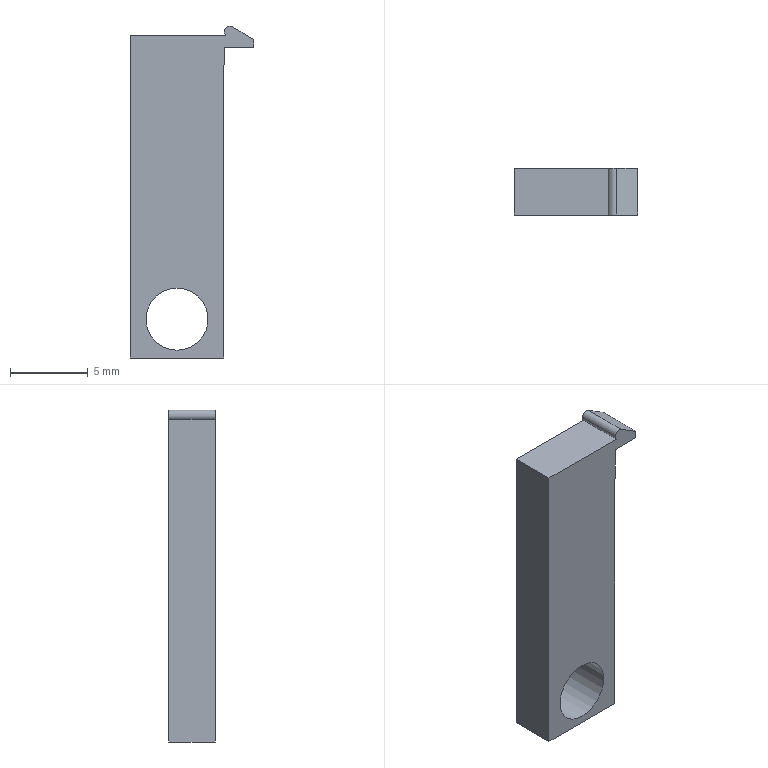Component | NX | SHEJI-WAIGUAN-3 | 1 solid | 12 faces | box 7.93 x 3 x 21.38 mm | volume 342 mm3 | plane 10 | cylinder 2 | commonest cylinder face diameters 0.707 x1 4 x1
STEP:
#1=CARTESIAN_POINT('',(0.,0.,0.));
#2=DIRECTION('',(0.,0.,1.));
#3=DIRECTION('',(1.,0.,0.));
#4=AXIS2_PLACEMENT_3D('',#1,#2,#3);
#5=CARTESIAN_POINT('',(-72.,-1.5,27.));
#6=VERTEX_POINT('',#5);
#7=CARTESIAN_POINT('',(-72.,-1.5,11.));
#8=VERTEX_POINT('',#7);
#9=CARTESIAN_POINT('',(-72.,-1.5,27.));
#10=DIRECTION('',(0.,0.,-1.));
#11=VECTOR('',#10,1.);
#12=LINE('',#9,#11);
#13=CARTESIAN_POINT('',(-72.,1.5,27.));
#14=DIRECTION('',(-1.,0.,0.));
#15=DIRECTION('',(0.,0.,-1.));
#16=AXIS2_PLACEMENT_3D('',#13,#14,#15);
#17=PLANE('',#16);
#18=CARTESIAN_POINT('',(0.,3.));
#19=DIRECTION('',(1.,0.));
#20=VECTOR('',#19,1.);
#21=LINE('',#18,#20);
#22=(GEOMETRIC_REPRESENTATION_CONTEXT(2)PARAMETRIC_REPRESENTATION_CONTEXT()REPRESENTATION_CONTEXT('',''));
#23=DEFINITIONAL_REPRESENTATION('',(#21),#22);
#24=PCURVE('',#17,#23);
#25=CARTESIAN_POINT('',(-71.606,-1.5,32.023));
#26=DIRECTION('',(0.,1.,0.));
#27=DIRECTION('',(0.,0.,-1.));
#28=AXIS2_PLACEMENT_3D('',#25,#26,#27);
#29=PLANE('',#28);
#30=CARTESIAN_POINT('',(5.023,0.3939));
#31=DIRECTION('',(1.,0.));
#32=VECTOR('',#31,1.);
#33=LINE('',#30,#32);
#34=(GEOMETRIC_REPRESENTATION_CONTEXT(2)PARAMETRIC_REPRESENTATION_CONTEXT()REPRESENTATION_CONTEXT('',''));
#35=DEFINITIONAL_REPRESENTATION('',(#33),#34);
#36=PCURVE('',#29,#35);
#37=SURFACE_CURVE('',#12,(#24,#36),.PCURVE_S1.);
#38=EDGE_CURVE('',#6,#8,#37,.T.);
#39=ORIENTED_EDGE('',*,*,#38,.T.);
#40=CARTESIAN_POINT('',(-72.,1.5,11.));
#41=VERTEX_POINT('',#40);
#42=CARTESIAN_POINT('',(-72.,1.5,11.));
#43=DIRECTION('',(0.,-1.,0.));
#44=VECTOR('',#43,1.);
#45=LINE('',#42,#44);
#46=CARTESIAN_POINT('',(16.,0.));
#47=DIRECTION('',(0.,1.));
#48=VECTOR('',#47,1.);
#49=LINE('',#46,#48);
#50=(GEOMETRIC_REPRESENTATION_CONTEXT(2)PARAMETRIC_REPRESENTATION_CONTEXT()REPRESENTATION_CONTEXT('',''));
#51=DEFINITIONAL_REPRESENTATION('',(#49),#50);
#52=PCURVE('',#17,#51);
#53=CARTESIAN_POINT('',(-72.,1.5,11.));
#54=DIRECTION('',(0.,0.,1.));
#55=DIRECTION('',(-1.,0.,0.));
#56=AXIS2_PLACEMENT_3D('',#53,#54,#55);
#57=PLANE('',#56);
#58=CARTESIAN_POINT('',(0.,0.));
#59=DIRECTION('',(0.,1.));
#60=VECTOR('',#59,1.);
#61=LINE('',#58,#60);
#62=(GEOMETRIC_REPRESENTATION_CONTEXT(2)PARAMETRIC_REPRESENTATION_CONTEXT()REPRESENTATION_CONTEXT('',''));
#63=DEFINITIONAL_REPRESENTATION('',(#61),#62);
#64=PCURVE('',#57,#63);
#65=SURFACE_CURVE('',#45,(#52,#64),.PCURVE_S1.);
#66=EDGE_CURVE('',#41,#8,#65,.T.);
#67=ORIENTED_EDGE('',*,*,#66,.F.);
#68=CARTESIAN_POINT('',(-72.,1.5,27.));
#69=VERTEX_POINT('',#68);
#70=CARTESIAN_POINT('',(-72.,1.5,27.));
#71=DIRECTION('',(0.,0.,-1.));
#72=VECTOR('',#71,1.);
#73=LINE('',#70,#72);
#74=CARTESIAN_POINT('',(0.,0.));
#75=DIRECTION('',(1.,0.));
#76=VECTOR('',#75,1.);
#77=LINE('',#74,#76);
#78=(GEOMETRIC_REPRESENTATION_CONTEXT(2)PARAMETRIC_REPRESENTATION_CONTEXT()REPRESENTATION_CONTEXT('',''));
#79=DEFINITIONAL_REPRESENTATION('',(#77),#78);
#80=PCURVE('',#17,#79);
#81=CARTESIAN_POINT('',(-71.606,1.5,32.023));
#82=DIRECTION('',(0.,1.,0.));
#83=DIRECTION('',(0.,0.,-1.));
#84=AXIS2_PLACEMENT_3D('',#81,#82,#83);
#85=PLANE('',#84);
#86=CARTESIAN_POINT('',(5.023,0.3939));
#87=DIRECTION('',(1.,0.));
#88=VECTOR('',#87,1.);
#89=LINE('',#86,#88);
#90=(GEOMETRIC_REPRESENTATION_CONTEXT(2)PARAMETRIC_REPRESENTATION_CONTEXT()REPRESENTATION_CONTEXT('',''));
#91=DEFINITIONAL_REPRESENTATION('',(#89),#90);
#92=PCURVE('',#85,#91);
#93=SURFACE_CURVE('',#73,(#80,#92),.PCURVE_S1.);
#94=EDGE_CURVE('',#69,#41,#93,.T.);
#95=ORIENTED_EDGE('',*,*,#94,.F.);
#96=CARTESIAN_POINT('',(-72.,1.5,27.));
#97=DIRECTION('',(0.,-1.,0.));
#98=VECTOR('',#97,1.);
#99=LINE('',#96,#98);
#100=CARTESIAN_POINT('',(0.,0.));
#101=DIRECTION('',(0.,1.));
#102=VECTOR('',#101,1.);
#103=LINE('',#100,#102);
#104=(GEOMETRIC_REPRESENTATION_CONTEXT(2)PARAMETRIC_REPRESENTATION_CONTEXT()REPRESENTATION_CONTEXT('',''));
#105=DEFINITIONAL_REPRESENTATION('',(#103),#104);
#106=PCURVE('',#17,#105);
#107=CARTESIAN_POINT('',(-71.968,1.5,31.));
#108=DIRECTION('',(-1.,0.,0.008057));
#109=DIRECTION('',(-0.008057,0.,-1.));
#110=AXIS2_PLACEMENT_3D('',#107,#108,#109);
#111=PLANE('',#110);
#112=CARTESIAN_POINT('',(4.,0.));
#113=DIRECTION('',(0.,1.));
#114=VECTOR('',#113,1.);
#115=LINE('',#112,#114);
#116=(GEOMETRIC_REPRESENTATION_CONTEXT(2)PARAMETRIC_REPRESENTATION_CONTEXT()REPRESENTATION_CONTEXT('',''));
#117=DEFINITIONAL_REPRESENTATION('',(#115),#116);
#118=PCURVE('',#111,#117);
#119=SURFACE_CURVE('',#99,(#106,#118),.PCURVE_S1.);
#120=EDGE_CURVE('',#69,#6,#119,.T.);
#121=ORIENTED_EDGE('',*,*,#120,.T.);
#122=EDGE_LOOP('',(#39,#67,#95,#121));
#123=FACE_BOUND('',#122,.T.);
#124=ADVANCED_FACE('',(#123),#17,.F.);
#125=CARTESIAN_POINT('',(-78.,-1.5,11.));
#126=VERTEX_POINT('',#125);
#127=CARTESIAN_POINT('',(-72.,-1.5,11.));
#128=DIRECTION('',(-1.,0.,0.));
#129=VECTOR('',#128,1.);
#130=LINE('',#127,#129);
#131=CARTESIAN_POINT('',(0.,3.));
#132=DIRECTION('',(1.,0.));
#133=VECTOR('',#132,1.);
#134=LINE('',#131,#133);
#135=(GEOMETRIC_REPRESENTATION_CONTEXT(2)PARAMETRIC_REPRESENTATION_CONTEXT()REPRESENTATION_CONTEXT('',''));
#136=DEFINITIONAL_REPRESENTATION('',(#134),#135);
#137=PCURVE('',#57,#136);
#138=CARTESIAN_POINT('',(21.023,0.3939));
#139=DIRECTION('',(0.,1.));
#140=VECTOR('',#139,1.);
#141=LINE('',#138,#140);
#142=(GEOMETRIC_REPRESENTATION_CONTEXT(2)PARAMETRIC_REPRESENTATION_CONTEXT()REPRESENTATION_CONTEXT('',''));
#143=DEFINITIONAL_REPRESENTATION('',(#141),#142);
#144=PCURVE('',#29,#143);
#145=SURFACE_CURVE('',#130,(#137,#144),.PCURVE_S1.);
#146=EDGE_CURVE('',#8,#126,#145,.T.);
#147=ORIENTED_EDGE('',*,*,#146,.T.);
#148=CARTESIAN_POINT('',(-78.,1.5,11.));
#149=VERTEX_POINT('',#148);
#150=CARTESIAN_POINT('',(-78.,1.5,11.));
#151=DIRECTION('',(0.,-1.,0.));
#152=VECTOR('',#151,1.);
#153=LINE('',#150,#152);
#154=CARTESIAN_POINT('',(6.,0.));
#155=DIRECTION('',(0.,1.));
#156=VECTOR('',#155,1.);
#157=LINE('',#154,#156);
#158=(GEOMETRIC_REPRESENTATION_CONTEXT(2)PARAMETRIC_REPRESENTATION_CONTEXT()REPRESENTATION_CONTEXT('',''));
#159=DEFINITIONAL_REPRESENTATION('',(#157),#158);
#160=PCURVE('',#57,#159);
#161=CARTESIAN_POINT('',(-78.,1.5,31.));
#162=DIRECTION('',(1.,0.,0.));
#163=DIRECTION('',(0.,0.,1.));
#164=AXIS2_PLACEMENT_3D('',#161,#162,#163);
#165=PLANE('',#164);
#166=CARTESIAN_POINT('',(-20.,0.));
#167=DIRECTION('',(0.,1.));
#168=VECTOR('',#167,1.);
#169=LINE('',#166,#168);
#170=(GEOMETRIC_REPRESENTATION_CONTEXT(2)PARAMETRIC_REPRESENTATION_CONTEXT()REPRESENTATION_CONTEXT('',''));
#171=DEFINITIONAL_REPRESENTATION('',(#169),#170);
#172=PCURVE('',#165,#171);
#173=SURFACE_CURVE('',#153,(#160,#172),.PCURVE_S1.);
#174=EDGE_CURVE('',#149,#126,#173,.T.);
#175=ORIENTED_EDGE('',*,*,#174,.F.);
#176=CARTESIAN_POINT('',(-72.,1.5,11.));
#177=DIRECTION('',(-1.,0.,0.));
#178=VECTOR('',#177,1.);
#179=LINE('',#176,#178);
#180=CARTESIAN_POINT('',(0.,0.));
#181=DIRECTION('',(1.,0.));
#182=VECTOR('',#181,1.);
#183=LINE('',#180,#182);
#184=(GEOMETRIC_REPRESENTATION_CONTEXT(2)PARAMETRIC_REPRESENTATION_CONTEXT()REPRESENTATION_CONTEXT('',''));
#185=DEFINITIONAL_REPRESENTATION('',(#183),#184);
#186=PCURVE('',#57,#185);
#187=CARTESIAN_POINT('',(21.023,0.3939));
#188=DIRECTION('',(0.,1.));
#189=VECTOR('',#188,1.);
#190=LINE('',#187,#189);
#191=(GEOMETRIC_REPRESENTATION_CONTEXT(2)PARAMETRIC_REPRESENTATION_CONTEXT()REPRESENTATION_CONTEXT('',''));
#192=DEFINITIONAL_REPRESENTATION('',(#190),#191);
#193=PCURVE('',#85,#192);
#194=SURFACE_CURVE('',#179,(#186,#193),.PCURVE_S1.);
#195=EDGE_CURVE('',#41,#149,#194,.T.);
#196=ORIENTED_EDGE('',*,*,#195,.F.);
#197=ORIENTED_EDGE('',*,*,#66,.T.);
#198=EDGE_LOOP('',(#147,#175,#196,#197));
#199=FACE_BOUND('',#198,.T.);
#200=ADVANCED_FACE('',(#199),#57,.F.);
#201=CARTESIAN_POINT('',(-78.,-1.5,31.776));
#202=VERTEX_POINT('',#201);
#203=CARTESIAN_POINT('',(-78.,-1.5,31.));
#204=DIRECTION('',(0.,0.,1.));
#205=VECTOR('',#204,1.);
#206=LINE('',#203,#205);
#207=CARTESIAN_POINT('',(0.,3.));
#208=DIRECTION('',(1.,0.));
#209=VECTOR('',#208,1.);
#210=LINE('',#207,#209);
#211=(GEOMETRIC_REPRESENTATION_CONTEXT(2)PARAMETRIC_REPRESENTATION_CONTEXT()REPRESENTATION_CONTEXT('',''));
#212=DEFINITIONAL_REPRESENTATION('',(#210),#211);
#213=PCURVE('',#165,#212);
#214=CARTESIAN_POINT('',(1.023,6.394));
#215=DIRECTION('',(-1.,0.));
#216=VECTOR('',#215,1.);
#217=LINE('',#214,#216);
#218=(GEOMETRIC_REPRESENTATION_CONTEXT(2)PARAMETRIC_REPRESENTATION_CONTEXT()REPRESENTATION_CONTEXT('',''));
#219=DEFINITIONAL_REPRESENTATION('',(#217),#218);
#220=PCURVE('',#29,#219);
#221=SURFACE_CURVE('',#206,(#213,#220),.PCURVE_S1.);
#222=EDGE_CURVE('',#126,#202,#221,.T.);
#223=ORIENTED_EDGE('',*,*,#222,.T.);
#224=CARTESIAN_POINT('',(-78.,1.5,31.776));
#225=VERTEX_POINT('',#224);
#226=CARTESIAN_POINT('',(-78.,1.5,31.776));
#227=DIRECTION('',(0.,-1.,0.));
#228=VECTOR('',#227,1.);
#229=LINE('',#226,#228);
#230=CARTESIAN_POINT('',(0.7762,0.));
#231=DIRECTION('',(0.,1.));
#232=VECTOR('',#231,1.);
#233=LINE('',#230,#232);
#234=(GEOMETRIC_REPRESENTATION_CONTEXT(2)PARAMETRIC_REPRESENTATION_CONTEXT()REPRESENTATION_CONTEXT('',''));
#235=DEFINITIONAL_REPRESENTATION('',(#233),#234);
#236=PCURVE('',#165,#235);
#237=CARTESIAN_POINT('',(-78.,1.5,31.776));
#238=DIRECTION('',(0.,0.,-1.));
#239=DIRECTION('',(1.,0.,0.));
#240=AXIS2_PLACEMENT_3D('',#237,#238,#239);
#241=PLANE('',#240);
#242=CARTESIAN_POINT('',(0.,0.));
#243=DIRECTION('',(0.,1.));
#244=VECTOR('',#243,1.);
#245=LINE('',#242,#244);
#246=(GEOMETRIC_REPRESENTATION_CONTEXT(2)PARAMETRIC_REPRESENTATION_CONTEXT()REPRESENTATION_CONTEXT('',''));
#247=DEFINITIONAL_REPRESENTATION('',(#245),#246);
#248=PCURVE('',#241,#247);
#249=SURFACE_CURVE('',#229,(#236,#248),.PCURVE_S1.);
#250=EDGE_CURVE('',#225,#202,#249,.T.);
#251=ORIENTED_EDGE('',*,*,#250,.F.);
#252=CARTESIAN_POINT('',(-78.,1.5,11.));
#253=DIRECTION('',(0.,0.,1.));
#254=VECTOR('',#253,1.);
#255=LINE('',#252,#254);
#256=CARTESIAN_POINT('',(-20.,0.));
#257=DIRECTION('',(1.,0.));
#258=VECTOR('',#257,1.);
#259=LINE('',#256,#258);
#260=(GEOMETRIC_REPRESENTATION_CONTEXT(2)PARAMETRIC_REPRESENTATION_CONTEXT()REPRESENTATION_CONTEXT('',''));
#261=DEFINITIONAL_REPRESENTATION('',(#259),#260);
#262=PCURVE('',#165,#261);
#263=CARTESIAN_POINT('',(21.023,6.394));
#264=DIRECTION('',(-1.,0.));
#265=VECTOR('',#264,1.);
#266=LINE('',#263,#265);
#267=(GEOMETRIC_REPRESENTATION_CONTEXT(2)PARAMETRIC_REPRESENTATION_CONTEXT()REPRESENTATION_CONTEXT('',''));
#268=DEFINITIONAL_REPRESENTATION('',(#266),#267);
#269=PCURVE('',#85,#268);
#270=SURFACE_CURVE('',#255,(#262,#269),.PCURVE_S1.);
#271=EDGE_CURVE('',#149,#225,#270,.T.);
#272=ORIENTED_EDGE('',*,*,#271,.F.);
#273=ORIENTED_EDGE('',*,*,#174,.T.);
#274=EDGE_LOOP('',(#223,#251,#272,#273));
#275=FACE_BOUND('',#274,.T.);
#276=ADVANCED_FACE('',(#275),#165,.F.);
#277=CARTESIAN_POINT('',(-71.859,-1.5,31.776));
#278=VERTEX_POINT('',#277);
#279=CARTESIAN_POINT('',(-78.,-1.5,31.776));
#280=DIRECTION('',(1.,0.,0.));
#281=VECTOR('',#280,1.);
#282=LINE('',#279,#281);
#283=CARTESIAN_POINT('',(0.,3.));
#284=DIRECTION('',(1.,0.));
#285=VECTOR('',#284,1.);
#286=LINE('',#283,#285);
#287=(GEOMETRIC_REPRESENTATION_CONTEXT(2)PARAMETRIC_REPRESENTATION_CONTEXT()REPRESENTATION_CONTEXT('',''));
#288=DEFINITIONAL_REPRESENTATION('',(#286),#287);
#289=PCURVE('',#241,#288);
#290=CARTESIAN_POINT('',(0.2472,6.394));
#291=DIRECTION('',(0.,-1.));
#292=VECTOR('',#291,1.);
#293=LINE('',#290,#292);
#294=(GEOMETRIC_REPRESENTATION_CONTEXT(2)PARAMETRIC_REPRESENTATION_CONTEXT()REPRESENTATION_CONTEXT('',''));
#295=DEFINITIONAL_REPRESENTATION('',(#293),#294);
#296=PCURVE('',#29,#295);
#297=SURFACE_CURVE('',#282,(#289,#296),.PCURVE_S1.);
#298=EDGE_CURVE('',#202,#278,#297,.T.);
#299=ORIENTED_EDGE('',*,*,#298,.T.);
#300=CARTESIAN_POINT('',(-71.859,1.5,31.776));
#301=VERTEX_POINT('',#300);
#302=CARTESIAN_POINT('',(-71.859,1.5,31.776));
#303=DIRECTION('',(0.,-1.,0.));
#304=VECTOR('',#303,1.);
#305=LINE('',#302,#304);
#306=CARTESIAN_POINT('',(6.141,-0.));
#307=DIRECTION('',(0.,1.));
#308=VECTOR('',#307,1.);
#309=LINE('',#306,#308);
#310=(GEOMETRIC_REPRESENTATION_CONTEXT(2)PARAMETRIC_REPRESENTATION_CONTEXT()REPRESENTATION_CONTEXT('',''));
#311=DEFINITIONAL_REPRESENTATION('',(#309),#310);
#312=PCURVE('',#241,#311);
#313=CARTESIAN_POINT('',(-71.606,1.5,32.023));
#314=DIRECTION('',(0.,-1.,0.));
#315=DIRECTION('',(0.,0.,1.));
#316=AXIS2_PLACEMENT_3D('',#313,#314,#315);
#317=CYLINDRICAL_SURFACE('',#316,0.3534);
#318=CARTESIAN_POINT('',(2.345,0.));
#319=DIRECTION('',(0.,1.));
#320=VECTOR('',#319,1.);
#321=LINE('',#318,#320);
#322=(GEOMETRIC_REPRESENTATION_CONTEXT(2)PARAMETRIC_REPRESENTATION_CONTEXT()REPRESENTATION_CONTEXT('',''));
#323=DEFINITIONAL_REPRESENTATION('',(#321),#322);
#324=PCURVE('',#317,#323);
#325=SURFACE_CURVE('',#305,(#312,#324),.PCURVE_S1.);
#326=EDGE_CURVE('',#301,#278,#325,.T.);
#327=ORIENTED_EDGE('',*,*,#326,.F.);
#328=CARTESIAN_POINT('',(-78.,1.5,31.776));
#329=DIRECTION('',(1.,0.,0.));
#330=VECTOR('',#329,1.);
#331=LINE('',#328,#330);
#332=CARTESIAN_POINT('',(0.,0.));
#333=DIRECTION('',(1.,0.));
#334=VECTOR('',#333,1.);
#335=LINE('',#332,#334);
#336=(GEOMETRIC_REPRESENTATION_CONTEXT(2)PARAMETRIC_REPRESENTATION_CONTEXT()REPRESENTATION_CONTEXT('',''));
#337=DEFINITIONAL_REPRESENTATION('',(#335),#336);
#338=PCURVE('',#241,#337);
#339=CARTESIAN_POINT('',(0.2472,6.394));
#340=DIRECTION('',(0.,-1.));
#341=VECTOR('',#340,1.);
#342=LINE('',#339,#341);
#343=(GEOMETRIC_REPRESENTATION_CONTEXT(2)PARAMETRIC_REPRESENTATION_CONTEXT()REPRESENTATION_CONTEXT('',''));
#344=DEFINITIONAL_REPRESENTATION('',(#342),#343);
#345=PCURVE('',#85,#344);
#346=SURFACE_CURVE('',#331,(#338,#345),.PCURVE_S1.);
#347=EDGE_CURVE('',#225,#301,#346,.T.);
#348=ORIENTED_EDGE('',*,*,#347,.F.);
#349=ORIENTED_EDGE('',*,*,#250,.T.);
#350=EDGE_LOOP('',(#299,#327,#348,#349));
#351=FACE_BOUND('',#350,.T.);
#352=ADVANCED_FACE('',(#351),#241,.F.);
#353=CARTESIAN_POINT('',(-71.421,-1.5,32.325));
#354=VERTEX_POINT('',#353);
#355=CARTESIAN_POINT('',(-71.606,-1.5,32.023));
#356=DIRECTION('',(0.,1.,0.));
#357=DIRECTION('',(-1.,0.,0.));
#358=AXIS2_PLACEMENT_3D('',#355,#356,#357);
#359=CIRCLE('',#358,0.3534);
#360=CARTESIAN_POINT('',(7.854,3.));
#361=DIRECTION('',(-1.,0.));
#362=VECTOR('',#361,1.);
#363=LINE('',#360,#362);
#364=(GEOMETRIC_REPRESENTATION_CONTEXT(2)PARAMETRIC_REPRESENTATION_CONTEXT()REPRESENTATION_CONTEXT('',''));
#365=DEFINITIONAL_REPRESENTATION('',(#363),#364);
#366=PCURVE('',#317,#365);
#367=CARTESIAN_POINT('',(0.,0.));
#368=DIRECTION('',(0.,1.));
#369=AXIS2_PLACEMENT_2D('',#367,#368);
#370=CIRCLE('',#369,0.3534);
#371=(GEOMETRIC_REPRESENTATION_CONTEXT(2)PARAMETRIC_REPRESENTATION_CONTEXT()REPRESENTATION_CONTEXT('',''));
#372=DEFINITIONAL_REPRESENTATION('',(#370),#371);
#373=PCURVE('',#29,#372);
#374=SURFACE_CURVE('',#359,(#366,#373),.PCURVE_S1.);
#375=EDGE_CURVE('',#278,#354,#374,.T.);
#376=ORIENTED_EDGE('',*,*,#375,.T.);
#377=CARTESIAN_POINT('',(-71.421,1.5,32.325));
#378=VERTEX_POINT('',#377);
#379=CARTESIAN_POINT('',(-71.421,1.5,32.325));
#380=DIRECTION('',(0.,-1.,0.));
#381=VECTOR('',#380,1.);
#382=LINE('',#379,#381);
#383=CARTESIAN_POINT('',(-0.5495,0.));
#384=DIRECTION('',(0.,1.));
#385=VECTOR('',#384,1.);
#386=LINE('',#383,#385);
#387=(GEOMETRIC_REPRESENTATION_CONTEXT(2)PARAMETRIC_REPRESENTATION_CONTEXT()REPRESENTATION_CONTEXT('',''));
#388=DEFINITIONAL_REPRESENTATION('',(#386),#387);
#389=PCURVE('',#317,#388);
#390=CARTESIAN_POINT('',(-71.421,1.5,32.325));
#391=DIRECTION('',(-0.5223,0.,-0.8528));
#392=DIRECTION('',(0.8528,0.,-0.5223));
#393=AXIS2_PLACEMENT_3D('',#390,#391,#392);
#394=PLANE('',#393);
#395=CARTESIAN_POINT('',(0.,0.));
#396=DIRECTION('',(0.,1.));
#397=VECTOR('',#396,1.);
#398=LINE('',#395,#397);
#399=(GEOMETRIC_REPRESENTATION_CONTEXT(2)PARAMETRIC_REPRESENTATION_CONTEXT()REPRESENTATION_CONTEXT('',''));
#400=DEFINITIONAL_REPRESENTATION('',(#398),#399);
#401=PCURVE('',#394,#400);
#402=SURFACE_CURVE('',#382,(#389,#401),.PCURVE_S1.);
#403=EDGE_CURVE('',#378,#354,#402,.T.);
#404=ORIENTED_EDGE('',*,*,#403,.F.);
#405=CARTESIAN_POINT('',(-71.606,1.5,32.023));
#406=DIRECTION('',(0.,1.,0.));
#407=DIRECTION('',(-1.,0.,0.));
#408=AXIS2_PLACEMENT_3D('',#405,#406,#407);
#409=CIRCLE('',#408,0.3534);
#410=CARTESIAN_POINT('',(7.854,0.));
#411=DIRECTION('',(-1.,0.));
#412=VECTOR('',#411,1.);
#413=LINE('',#410,#412);
#414=(GEOMETRIC_REPRESENTATION_CONTEXT(2)PARAMETRIC_REPRESENTATION_CONTEXT()REPRESENTATION_CONTEXT('',''));
#415=DEFINITIONAL_REPRESENTATION('',(#413),#414);
#416=PCURVE('',#317,#415);
#417=CARTESIAN_POINT('',(0.,0.));
#418=DIRECTION('',(0.,1.));
#419=AXIS2_PLACEMENT_2D('',#417,#418);
#420=CIRCLE('',#419,0.3534);
#421=(GEOMETRIC_REPRESENTATION_CONTEXT(2)PARAMETRIC_REPRESENTATION_CONTEXT()REPRESENTATION_CONTEXT('',''));
#422=DEFINITIONAL_REPRESENTATION('',(#420),#421);
#423=PCURVE('',#85,#422);
#424=SURFACE_CURVE('',#409,(#416,#423),.PCURVE_S1.);
#425=EDGE_CURVE('',#301,#378,#424,.T.);
#426=ORIENTED_EDGE('',*,*,#425,.F.);
#427=ORIENTED_EDGE('',*,*,#326,.T.);
#428=EDGE_LOOP('',(#376,#404,#426,#427));
#429=FACE_BOUND('',#428,.T.);
#430=ADVANCED_FACE('',(#429),#317,.T.);
#431=CARTESIAN_POINT('',(-70.075,-1.5,31.5));
#432=VERTEX_POINT('',#431);
#433=CARTESIAN_POINT('',(-71.421,-1.5,32.325));
#434=DIRECTION('',(0.8528,-0.,-0.5223));
#435=VECTOR('',#434,1.);
#436=LINE('',#433,#435);
#437=CARTESIAN_POINT('',(0.,3.));
#438=DIRECTION('',(1.,0.));
#439=VECTOR('',#438,1.);
#440=LINE('',#437,#439);
#441=(GEOMETRIC_REPRESENTATION_CONTEXT(2)PARAMETRIC_REPRESENTATION_CONTEXT()REPRESENTATION_CONTEXT('',''));
#442=DEFINITIONAL_REPRESENTATION('',(#440),#441);
#443=PCURVE('',#394,#442);
#444=CARTESIAN_POINT('',(-0.3014,-0.1846));
#445=DIRECTION('',(0.5223,-0.8528));
#446=VECTOR('',#445,1.);
#447=LINE('',#444,#446);
#448=(GEOMETRIC_REPRESENTATION_CONTEXT(2)PARAMETRIC_REPRESENTATION_CONTEXT()REPRESENTATION_CONTEXT('',''));
#449=DEFINITIONAL_REPRESENTATION('',(#447),#448);
#450=PCURVE('',#29,#449);
#451=SURFACE_CURVE('',#436,(#443,#450),.PCURVE_S1.);
#452=EDGE_CURVE('',#354,#432,#451,.T.);
#453=ORIENTED_EDGE('',*,*,#452,.T.);
#454=CARTESIAN_POINT('',(-70.075,1.5,31.5));
#455=VERTEX_POINT('',#454);
#456=CARTESIAN_POINT('',(-70.075,1.5,31.5));
#457=DIRECTION('',(0.,-1.,0.));
#458=VECTOR('',#457,1.);
#459=LINE('',#456,#458);
#460=CARTESIAN_POINT('',(1.579,0.));
#461=DIRECTION('',(0.,1.));
#462=VECTOR('',#461,1.);
#463=LINE('',#460,#462);
#464=(GEOMETRIC_REPRESENTATION_CONTEXT(2)PARAMETRIC_REPRESENTATION_CONTEXT()REPRESENTATION_CONTEXT('',''));
#465=DEFINITIONAL_REPRESENTATION('',(#463),#464);
#466=PCURVE('',#394,#465);
#467=CARTESIAN_POINT('',(-70.075,1.5,31.5));
#468=DIRECTION('',(-1.,0.,-0.));
#469=DIRECTION('',(0.,0.,-1.));
#470=AXIS2_PLACEMENT_3D('',#467,#468,#469);
#471=PLANE('',#470);
#472=CARTESIAN_POINT('',(0.,0.));
#473=DIRECTION('',(0.,1.));
#474=VECTOR('',#473,1.);
#475=LINE('',#472,#474);
#476=(GEOMETRIC_REPRESENTATION_CONTEXT(2)PARAMETRIC_REPRESENTATION_CONTEXT()REPRESENTATION_CONTEXT('',''));
#477=DEFINITIONAL_REPRESENTATION('',(#475),#476);
#478=PCURVE('',#471,#477);
#479=SURFACE_CURVE('',#459,(#466,#478),.PCURVE_S1.);
#480=EDGE_CURVE('',#455,#432,#479,.T.);
#481=ORIENTED_EDGE('',*,*,#480,.F.);
#482=CARTESIAN_POINT('',(-71.421,1.5,32.325));
#483=DIRECTION('',(0.8528,-0.,-0.5223));
#484=VECTOR('',#483,1.);
#485=LINE('',#482,#484);
#486=CARTESIAN_POINT('',(0.,0.));
#487=DIRECTION('',(1.,0.));
#488=VECTOR('',#487,1.);
#489=LINE('',#486,#488);
#490=(GEOMETRIC_REPRESENTATION_CONTEXT(2)PARAMETRIC_REPRESENTATION_CONTEXT()REPRESENTATION_CONTEXT('',''));
#491=DEFINITIONAL_REPRESENTATION('',(#489),#490);
#492=PCURVE('',#394,#491);
#493=CARTESIAN_POINT('',(-0.3014,-0.1846));
#494=DIRECTION('',(0.5223,-0.8528));
#495=VECTOR('',#494,1.);
#496=LINE('',#493,#495);
#497=(GEOMETRIC_REPRESENTATION_CONTEXT(2)PARAMETRIC_REPRESENTATION_CONTEXT()REPRESENTATION_CONTEXT('',''));
#498=DEFINITIONAL_REPRESENTATION('',(#496),#497);
#499=PCURVE('',#85,#498);
#500=SURFACE_CURVE('',#485,(#492,#499),.PCURVE_S1.);
#501=EDGE_CURVE('',#378,#455,#500,.T.);
#502=ORIENTED_EDGE('',*,*,#501,.F.);
#503=ORIENTED_EDGE('',*,*,#403,.T.);
#504=EDGE_LOOP('',(#453,#481,#502,#503));
#505=FACE_BOUND('',#504,.T.);
#506=ADVANCED_FACE('',(#505),#394,.F.);
#507=CARTESIAN_POINT('',(-70.075,-1.5,31.));
#508=VERTEX_POINT('',#507);
#509=CARTESIAN_POINT('',(-70.075,-1.5,31.5));
#510=DIRECTION('',(0.,0.,-1.));
#511=VECTOR('',#510,1.);
#512=LINE('',#509,#511);
#513=CARTESIAN_POINT('',(0.,3.));
#514=DIRECTION('',(1.,-0.));
#515=VECTOR('',#514,1.);
#516=LINE('',#513,#515);
#517=(GEOMETRIC_REPRESENTATION_CONTEXT(2)PARAMETRIC_REPRESENTATION_CONTEXT()REPRESENTATION_CONTEXT('',''));
#518=DEFINITIONAL_REPRESENTATION('',(#516),#517);
#519=PCURVE('',#471,#518);
#520=CARTESIAN_POINT('',(0.5234,-1.531));
#521=DIRECTION('',(1.,-0.));
#522=VECTOR('',#521,1.);
#523=LINE('',#520,#522);
#524=(GEOMETRIC_REPRESENTATION_CONTEXT(2)PARAMETRIC_REPRESENTATION_CONTEXT()REPRESENTATION_CONTEXT('',''));
#525=DEFINITIONAL_REPRESENTATION('',(#523),#524);
#526=PCURVE('',#29,#525);
#527=SURFACE_CURVE('',#512,(#519,#526),.PCURVE_S1.);
#528=EDGE_CURVE('',#432,#508,#527,.T.);
#529=ORIENTED_EDGE('',*,*,#528,.T.);
#530=CARTESIAN_POINT('',(-70.075,1.5,31.));
#531=VERTEX_POINT('',#530);
#532=CARTESIAN_POINT('',(-70.075,1.5,31.));
#533=DIRECTION('',(0.,-1.,0.));
#534=VECTOR('',#533,1.);
#535=LINE('',#532,#534);
#536=CARTESIAN_POINT('',(0.5,0.));
#537=DIRECTION('',(0.,1.));
#538=VECTOR('',#537,1.);
#539=LINE('',#536,#538);
#540=(GEOMETRIC_REPRESENTATION_CONTEXT(2)PARAMETRIC_REPRESENTATION_CONTEXT()REPRESENTATION_CONTEXT('',''));
#541=DEFINITIONAL_REPRESENTATION('',(#539),#540);
#542=PCURVE('',#471,#541);
#543=CARTESIAN_POINT('',(-70.075,1.5,31.));
#544=DIRECTION('',(-0.,0.,1.));
#545=DIRECTION('',(-1.,0.,-0.));
#546=AXIS2_PLACEMENT_3D('',#543,#544,#545);
#547=PLANE('',#546);
#548=CARTESIAN_POINT('',(0.,0.));
#549=DIRECTION('',(0.,1.));
#550=VECTOR('',#549,1.);
#551=LINE('',#548,#550);
#552=(GEOMETRIC_REPRESENTATION_CONTEXT(2)PARAMETRIC_REPRESENTATION_CONTEXT()REPRESENTATION_CONTEXT('',''));
#553=DEFINITIONAL_REPRESENTATION('',(#551),#552);
#554=PCURVE('',#547,#553);
#555=SURFACE_CURVE('',#535,(#542,#554),.PCURVE_S1.);
#556=EDGE_CURVE('',#531,#508,#555,.T.);
#557=ORIENTED_EDGE('',*,*,#556,.F.);
#558=CARTESIAN_POINT('',(-70.075,1.5,31.5));
#559=DIRECTION('',(0.,0.,-1.));
#560=VECTOR('',#559,1.);
#561=LINE('',#558,#560);
#562=CARTESIAN_POINT('',(0.,0.));
#563=DIRECTION('',(1.,-0.));
#564=VECTOR('',#563,1.);
#565=LINE('',#562,#564);
#566=(GEOMETRIC_REPRESENTATION_CONTEXT(2)PARAMETRIC_REPRESENTATION_CONTEXT()REPRESENTATION_CONTEXT('',''));
#567=DEFINITIONAL_REPRESENTATION('',(#565),#566);
#568=PCURVE('',#471,#567);
#569=CARTESIAN_POINT('',(0.5234,-1.531));
#570=DIRECTION('',(1.,-0.));
#571=VECTOR('',#570,1.);
#572=LINE('',#569,#571);
#573=(GEOMETRIC_REPRESENTATION_CONTEXT(2)PARAMETRIC_REPRESENTATION_CONTEXT()REPRESENTATION_CONTEXT('',''));
#574=DEFINITIONAL_REPRESENTATION('',(#572),#573);
#575=PCURVE('',#85,#574);
#576=SURFACE_CURVE('',#561,(#568,#575),.PCURVE_S1.);
#577=EDGE_CURVE('',#455,#531,#576,.T.);
#578=ORIENTED_EDGE('',*,*,#577,.F.);
#579=ORIENTED_EDGE('',*,*,#480,.T.);
#580=EDGE_LOOP('',(#529,#557,#578,#579));
#581=FACE_BOUND('',#580,.T.);
#582=ADVANCED_FACE('',(#581),#471,.F.);
#583=CARTESIAN_POINT('',(-71.968,-1.5,31.));
#584=VERTEX_POINT('',#583);
#585=CARTESIAN_POINT('',(-70.075,-1.5,31.));
#586=DIRECTION('',(-1.,-0.,-0.));
#587=VECTOR('',#586,1.);
#588=LINE('',#585,#587);
#589=CARTESIAN_POINT('',(0.,3.));
#590=DIRECTION('',(1.,0.));
#591=VECTOR('',#590,1.);
#592=LINE('',#589,#591);
#593=(GEOMETRIC_REPRESENTATION_CONTEXT(2)PARAMETRIC_REPRESENTATION_CONTEXT()REPRESENTATION_CONTEXT('',''));
#594=DEFINITIONAL_REPRESENTATION('',(#592),#593);
#595=PCURVE('',#547,#594);
#596=CARTESIAN_POINT('',(1.023,-1.531));
#597=DIRECTION('',(0.,1.));
#598=VECTOR('',#597,1.);
#599=LINE('',#596,#598);
#600=(GEOMETRIC_REPRESENTATION_CONTEXT(2)PARAMETRIC_REPRESENTATION_CONTEXT()REPRESENTATION_CONTEXT('',''));
#601=DEFINITIONAL_REPRESENTATION('',(#599),#600);
#602=PCURVE('',#29,#601);
#603=SURFACE_CURVE('',#588,(#595,#602),.PCURVE_S1.);
#604=EDGE_CURVE('',#508,#584,#603,.T.);
#605=ORIENTED_EDGE('',*,*,#604,.T.);
#606=CARTESIAN_POINT('',(-71.968,1.5,31.));
#607=VERTEX_POINT('',#606);
#608=CARTESIAN_POINT('',(-71.968,1.5,31.));
#609=DIRECTION('',(0.,-1.,0.));
#610=VECTOR('',#609,1.);
#611=LINE('',#608,#610);
#612=CARTESIAN_POINT('',(1.893,0.));
#613=DIRECTION('',(0.,1.));
#614=VECTOR('',#613,1.);
#615=LINE('',#612,#614);
#616=(GEOMETRIC_REPRESENTATION_CONTEXT(2)PARAMETRIC_REPRESENTATION_CONTEXT()REPRESENTATION_CONTEXT('',''));
#617=DEFINITIONAL_REPRESENTATION('',(#615),#616);
#618=PCURVE('',#547,#617);
#619=CARTESIAN_POINT('',(0.,0.));
#620=DIRECTION('',(0.,1.));
#621=VECTOR('',#620,1.);
#622=LINE('',#619,#621);
#623=(GEOMETRIC_REPRESENTATION_CONTEXT(2)PARAMETRIC_REPRESENTATION_CONTEXT()REPRESENTATION_CONTEXT('',''));
#624=DEFINITIONAL_REPRESENTATION('',(#622),#623);
#625=PCURVE('',#111,#624);
#626=SURFACE_CURVE('',#611,(#618,#625),.PCURVE_S1.);
#627=EDGE_CURVE('',#607,#584,#626,.T.);
#628=ORIENTED_EDGE('',*,*,#627,.F.);
#629=CARTESIAN_POINT('',(-70.075,1.5,31.));
#630=DIRECTION('',(-1.,-0.,-0.));
#631=VECTOR('',#630,1.);
#632=LINE('',#629,#631);
#633=CARTESIAN_POINT('',(0.,0.));
#634=DIRECTION('',(1.,0.));
#635=VECTOR('',#634,1.);
#636=LINE('',#633,#635);
#637=(GEOMETRIC_REPRESENTATION_CONTEXT(2)PARAMETRIC_REPRESENTATION_CONTEXT()REPRESENTATION_CONTEXT('',''));
#638=DEFINITIONAL_REPRESENTATION('',(#636),#637);
#639=PCURVE('',#547,#638);
#640=CARTESIAN_POINT('',(1.023,-1.531));
#641=DIRECTION('',(0.,1.));
#642=VECTOR('',#641,1.);
#643=LINE('',#640,#642);
#644=(GEOMETRIC_REPRESENTATION_CONTEXT(2)PARAMETRIC_REPRESENTATION_CONTEXT()REPRESENTATION_CONTEXT('',''));
#645=DEFINITIONAL_REPRESENTATION('',(#643),#644);
#646=PCURVE('',#85,#645);
#647=SURFACE_CURVE('',#632,(#639,#646),.PCURVE_S1.);
#648=EDGE_CURVE('',#531,#607,#647,.T.);
#649=ORIENTED_EDGE('',*,*,#648,.F.);
#650=ORIENTED_EDGE('',*,*,#556,.T.);
#651=EDGE_LOOP('',(#605,#628,#649,#650));
#652=FACE_BOUND('',#651,.T.);
#653=ADVANCED_FACE('',(#652),#547,.F.);
#654=CARTESIAN_POINT('',(-71.968,-1.5,31.));
#655=DIRECTION('',(-0.008057,-0.,-1.));
#656=VECTOR('',#655,1.);
#657=LINE('',#654,#656);
#658=CARTESIAN_POINT('',(0.,3.));
#659=DIRECTION('',(1.,0.));
#660=VECTOR('',#659,1.);
#661=LINE('',#658,#660);
#662=(GEOMETRIC_REPRESENTATION_CONTEXT(2)PARAMETRIC_REPRESENTATION_CONTEXT()REPRESENTATION_CONTEXT('',''));
#663=DEFINITIONAL_REPRESENTATION('',(#661),#662);
#664=PCURVE('',#111,#663);
#665=CARTESIAN_POINT('',(1.023,0.3617));
#666=DIRECTION('',(1.,0.008057));
#667=VECTOR('',#666,1.);
#668=LINE('',#665,#667);
#669=(GEOMETRIC_REPRESENTATION_CONTEXT(2)PARAMETRIC_REPRESENTATION_CONTEXT()REPRESENTATION_CONTEXT('',''));
#670=DEFINITIONAL_REPRESENTATION('',(#668),#669);
#671=PCURVE('',#29,#670);
#672=SURFACE_CURVE('',#657,(#664,#671),.PCURVE_S1.);
#673=EDGE_CURVE('',#584,#6,#672,.T.);
#674=ORIENTED_EDGE('',*,*,#673,.T.);
#675=ORIENTED_EDGE('',*,*,#120,.F.);
#676=CARTESIAN_POINT('',(-71.968,1.5,31.));
#677=DIRECTION('',(-0.008057,-0.,-1.));
#678=VECTOR('',#677,1.);
#679=LINE('',#676,#678);
#680=CARTESIAN_POINT('',(0.,0.));
#681=DIRECTION('',(1.,0.));
#682=VECTOR('',#681,1.);
#683=LINE('',#680,#682);
#684=(GEOMETRIC_REPRESENTATION_CONTEXT(2)PARAMETRIC_REPRESENTATION_CONTEXT()REPRESENTATION_CONTEXT('',''));
#685=DEFINITIONAL_REPRESENTATION('',(#683),#684);
#686=PCURVE('',#111,#685);
#687=CARTESIAN_POINT('',(1.023,0.3617));
#688=DIRECTION('',(1.,0.008057));
#689=VECTOR('',#688,1.);
#690=LINE('',#687,#689);
#691=(GEOMETRIC_REPRESENTATION_CONTEXT(2)PARAMETRIC_REPRESENTATION_CONTEXT()REPRESENTATION_CONTEXT('',''));
#692=DEFINITIONAL_REPRESENTATION('',(#690),#691);
#693=PCURVE('',#85,#692);
#694=SURFACE_CURVE('',#679,(#686,#693),.PCURVE_S1.);
#695=EDGE_CURVE('',#607,#69,#694,.T.);
#696=ORIENTED_EDGE('',*,*,#695,.F.);
#697=ORIENTED_EDGE('',*,*,#627,.T.);
#698=EDGE_LOOP('',(#674,#675,#696,#697));
#699=FACE_BOUND('',#698,.T.);
#700=ADVANCED_FACE('',(#699),#111,.F.);
#701=CARTESIAN_POINT('',(-75.,1.5,11.5));
#702=VERTEX_POINT('',#701);
#703=CARTESIAN_POINT('',(-75.,1.5,13.5));
#704=DIRECTION('',(0.,-1.,0.));
#705=DIRECTION('',(0.,0.,-1.));
#706=AXIS2_PLACEMENT_3D('',#703,#704,#705);
#707=CIRCLE('',#706,2.);
#708=CARTESIAN_POINT('',(20.523,3.394));
#709=CARTESIAN_POINT('',(20.523,-0.07016));
#710=CARTESIAN_POINT('',(17.523,1.662));
#711=CARTESIAN_POINT('',(14.523,3.394));
#712=CARTESIAN_POINT('',(17.523,5.126));
#713=CARTESIAN_POINT('',(20.523,6.858));
#714=CARTESIAN_POINT('',(20.523,3.394));
#715=(BOUNDED_CURVE()B_SPLINE_CURVE(2,(#708,#709,#710,#711,#712,#713,#714),.UNSPECIFIED.,.T.,.F.)B_SPLINE_CURVE_WITH_KNOTS((1,2,2,2,2,1),(-2.094,0.,2.094,4.189,6.283,8.378),.UNSPECIFIED.)CURVE()GEOMETRIC_REPRESENTATION_ITEM()RATIONAL_B_SPLINE_CURVE((1.,0.5,1.,0.5,1.,0.5,1.))REPRESENTATION_ITEM(''));
#716=(GEOMETRIC_REPRESENTATION_CONTEXT(2)PARAMETRIC_REPRESENTATION_CONTEXT()REPRESENTATION_CONTEXT('',''));
#717=DEFINITIONAL_REPRESENTATION('',(#715),#716);
#718=PCURVE('',#85,#717);
#719=CARTESIAN_POINT('',(-75.,-7.7,13.5));
#720=DIRECTION('',(0.,1.,0.));
#721=DIRECTION('',(0.,0.,-1.));
#722=AXIS2_PLACEMENT_3D('',#719,#720,#721);
#723=CYLINDRICAL_SURFACE('',#722,2.);
#724=CARTESIAN_POINT('',(6.283,9.2));
#725=DIRECTION('',(-1.,0.));
#726=VECTOR('',#725,1.);
#727=LINE('',#724,#726);
#728=(GEOMETRIC_REPRESENTATION_CONTEXT(2)PARAMETRIC_REPRESENTATION_CONTEXT()REPRESENTATION_CONTEXT('',''));
#729=DEFINITIONAL_REPRESENTATION('',(#727),#728);
#730=PCURVE('',#723,#729);
#731=SURFACE_CURVE('',#707,(#718,#730),.PCURVE_S1.);
#732=EDGE_CURVE('',#702,#702,#731,.T.);
#733=ORIENTED_EDGE('',*,*,#732,.T.);
#734=EDGE_LOOP('',(#733));
#735=FACE_BOUND('',#734,.T.);
#736=ORIENTED_EDGE('',*,*,#94,.T.);
#737=ORIENTED_EDGE('',*,*,#195,.T.);
#738=ORIENTED_EDGE('',*,*,#271,.T.);
#739=ORIENTED_EDGE('',*,*,#347,.T.);
#740=ORIENTED_EDGE('',*,*,#425,.T.);
#741=ORIENTED_EDGE('',*,*,#501,.T.);
#742=ORIENTED_EDGE('',*,*,#577,.T.);
#743=ORIENTED_EDGE('',*,*,#648,.T.);
#744=ORIENTED_EDGE('',*,*,#695,.T.);
#745=EDGE_LOOP('',(#736,#737,#738,#739,#740,#741,#742,#743,#744));
#746=FACE_BOUND('',#745,.T.);
#747=ADVANCED_FACE('',(#735,#746),#85,.T.);
#748=CARTESIAN_POINT('',(-75.,-1.5,11.5));
#749=VERTEX_POINT('',#748);
#750=CARTESIAN_POINT('',(-75.,-1.5,13.5));
#751=DIRECTION('',(0.,-1.,0.));
#752=DIRECTION('',(0.,0.,-1.));
#753=AXIS2_PLACEMENT_3D('',#750,#751,#752);
#754=CIRCLE('',#753,2.);
#755=CARTESIAN_POINT('',(20.523,3.394));
#756=CARTESIAN_POINT('',(20.523,-0.07016));
#757=CARTESIAN_POINT('',(17.523,1.662));
#758=CARTESIAN_POINT('',(14.523,3.394));
#759=CARTESIAN_POINT('',(17.523,5.126));
#760=CARTESIAN_POINT('',(20.523,6.858));
#761=CARTESIAN_POINT('',(20.523,3.394));
#762=(BOUNDED_CURVE()B_SPLINE_CURVE(2,(#755,#756,#757,#758,#759,#760,#761),.UNSPECIFIED.,.T.,.F.)B_SPLINE_CURVE_WITH_KNOTS((1,2,2,2,2,1),(-2.094,0.,2.094,4.189,6.283,8.378),.UNSPECIFIED.)CURVE()GEOMETRIC_REPRESENTATION_ITEM()RATIONAL_B_SPLINE_CURVE((1.,0.5,1.,0.5,1.,0.5,1.))REPRESENTATION_ITEM(''));
#763=(GEOMETRIC_REPRESENTATION_CONTEXT(2)PARAMETRIC_REPRESENTATION_CONTEXT()REPRESENTATION_CONTEXT('',''));
#764=DEFINITIONAL_REPRESENTATION('',(#762),#763);
#765=PCURVE('',#29,#764);
#766=CARTESIAN_POINT('',(6.283,6.2));
#767=DIRECTION('',(-1.,0.));
#768=VECTOR('',#767,1.);
#769=LINE('',#766,#768);
#770=(GEOMETRIC_REPRESENTATION_CONTEXT(2)PARAMETRIC_REPRESENTATION_CONTEXT()REPRESENTATION_CONTEXT('',''));
#771=DEFINITIONAL_REPRESENTATION('',(#769),#770);
#772=PCURVE('',#723,#771);
#773=SURFACE_CURVE('',#754,(#765,#772),.PCURVE_S1.);
#774=EDGE_CURVE('',#749,#749,#773,.T.);
#775=ORIENTED_EDGE('',*,*,#774,.F.);
#776=EDGE_LOOP('',(#775));
#777=FACE_BOUND('',#776,.T.);
#778=ORIENTED_EDGE('',*,*,#38,.F.);
#779=ORIENTED_EDGE('',*,*,#673,.F.);
#780=ORIENTED_EDGE('',*,*,#604,.F.);
#781=ORIENTED_EDGE('',*,*,#528,.F.);
#782=ORIENTED_EDGE('',*,*,#452,.F.);
#783=ORIENTED_EDGE('',*,*,#375,.F.);
#784=ORIENTED_EDGE('',*,*,#298,.F.);
#785=ORIENTED_EDGE('',*,*,#222,.F.);
#786=ORIENTED_EDGE('',*,*,#146,.F.);
#787=EDGE_LOOP('',(#778,#779,#780,#781,#782,#783,#784,#785,#786));
#788=FACE_BOUND('',#787,.T.);
#789=ADVANCED_FACE('',(#777,#788),#29,.F.);
#790=ORIENTED_EDGE('',*,*,#732,.T.);
#791=CARTESIAN_POINT('',(-75.,-1.5,11.5));
#792=CARTESIAN_POINT('',(-75.,1.5,11.5));
#793=B_SPLINE_CURVE_WITH_KNOTS('',1,(#791,#792),.UNSPECIFIED.,.F.,.F.,(2,2),(6.2,9.2),.PIECEWISE_BEZIER_KNOTS.);
#794=CARTESIAN_POINT('',(0.,0.));
#795=DIRECTION('',(0.,1.));
#796=VECTOR('',#795,1.);
#797=LINE('',#794,#796);
#798=(GEOMETRIC_REPRESENTATION_CONTEXT(2)PARAMETRIC_REPRESENTATION_CONTEXT()REPRESENTATION_CONTEXT('',''));
#799=DEFINITIONAL_REPRESENTATION('',(#797),#798);
#800=PCURVE('',#723,#799);
#801=CARTESIAN_POINT('',(6.283,0.));
#802=DIRECTION('',(0.,1.));
#803=VECTOR('',#802,1.);
#804=LINE('',#801,#803);
#805=(GEOMETRIC_REPRESENTATION_CONTEXT(2)PARAMETRIC_REPRESENTATION_CONTEXT()REPRESENTATION_CONTEXT('',''));
#806=DEFINITIONAL_REPRESENTATION('',(#804),#805);
#807=PCURVE('',#723,#806);
#808=SEAM_CURVE('',#793,(#800,#807),.PCURVE_S1.);
#809=EDGE_CURVE('',#749,#702,#808,.T.);
#810=ORIENTED_EDGE('',*,*,#809,.F.);
#811=ORIENTED_EDGE('',*,*,#774,.F.);
#812=ORIENTED_EDGE('',*,*,#809,.T.);
#813=EDGE_LOOP('',(#790,#810,#811,#812));
#814=FACE_BOUND('',#813,.F.);
#815=ADVANCED_FACE('',(#814),#723,.F.);
#816=CLOSED_SHELL('',(#124,#200,#276,#352,#430,#506,#582,#653,#700,#747,#789,#815));
#817=MANIFOLD_SOLID_BREP('',#816);
#818=(LENGTH_UNIT()NAMED_UNIT(*)SI_UNIT(.MILLI.,.METRE.));
#819=UNCERTAINTY_MEASURE_WITH_UNIT(LENGTH_MEASURE(0.000001),#818,'','');
#820=(NAMED_UNIT(*)PLANE_ANGLE_UNIT()SI_UNIT($,.RADIAN.));
#821=(NAMED_UNIT(*)SI_UNIT($,.STERADIAN.)SOLID_ANGLE_UNIT());
#822=(GEOMETRIC_REPRESENTATION_CONTEXT(3)GLOBAL_UNCERTAINTY_ASSIGNED_CONTEXT((#819))GLOBAL_UNIT_ASSIGNED_CONTEXT((#818,#820,#821))REPRESENTATION_CONTEXT('',''));
#823=ADVANCED_BREP_SHAPE_REPRESENTATION('',(#4,#817),#822);